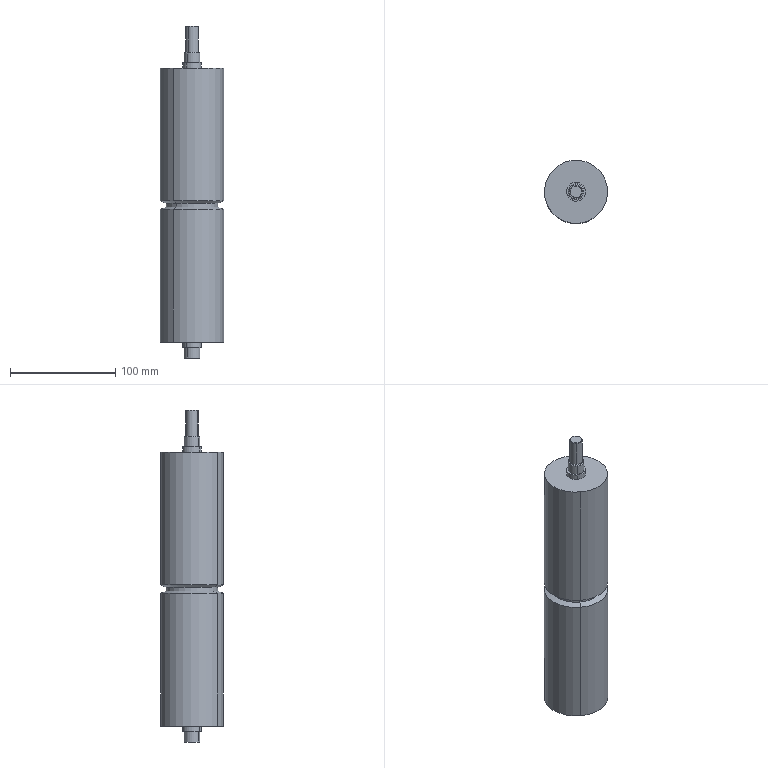Component | SolidWorks | LD101-02--Q1024-Q1-2-1 | 1 solid | 31 faces | box 60 x 60 x 315 mm | volume 738446 mm3 | cylinder 16 | cone 8 | plane 7 | commonest cylinder face diameters 60 x4 18 x4 15 x4 49 x2 12 x2 | material 45
build123d program:
from build123d import *

# Parameters (mm, degrees)
SKETCH1_R           = 30
SKETCH1_R_2         = 25
EXTRUDE_THIN1_DEPTH = 130
BOSS_EXTRUDE1_START = -260
SKETCH2_R           = 25
BOSS_EXTRUDE1_DEPTH = 260
SKETCH3_R           = 9
BOSS_EXTRUDE2_DEPTH = 5
SKETCH5_R           = 7.5
BOSS_EXTRUDE4_DEPTH = 10
BOSS_EXTRUDE5_START = 10
SKETCH6_R           = 7.5
BOSS_EXTRUDE5_DEPTH = 10
CHAMFER4_SIZE       = 0.6
SKETCH7_R           = 6
BOSS_EXTRUDE6_DEPTH = 25
CHAMFER3_SIZE       = 0.6


with BuildPart() as part:
    # Sketch1 → Extrude-Thin1 (new, symmetric)
    with BuildSketch(Plane.XY):
        Circle(SKETCH1_R)
        Circle(SKETCH1_R_2, mode=Mode.SUBTRACT)
    extrude(amount=EXTRUDE_THIN1_DEPTH, both=True)

    # Sketch2 → Boss-Extrude1 (add)
    with BuildSketch(Plane.XY.offset(130).offset(BOSS_EXTRUDE1_START)):
        Circle(SKETCH2_R)
    extrude(amount=BOSS_EXTRUDE1_DEPTH)

    # Sketch3 → Boss-Extrude2 (add)
    with BuildSketch(Plane.XY.offset(130)):
        Circle(SKETCH3_R)
    extrude(amount=BOSS_EXTRUDE2_DEPTH)

    # Mirror2: part across plane


with BuildPart() as part_1:
    add(part.part)
    add(part.part.mirror(Plane.XY))

    # Sketch5 → Boss-Extrude4 (add)
    with BuildSketch(Plane.XY.offset(135)):
        Circle(SKETCH5_R)
    extrude(amount=BOSS_EXTRUDE4_DEPTH)

    # Sketch6 → Boss-Extrude5 (add)
    with BuildSketch(Plane(origin=(0, 0, -135), x_dir=(-1, 0, 0), z_dir=(0, 0, -1)).offset(BOSS_EXTRUDE5_START)):
        with Locations(Location((0, 0, 0), (0, 0, 180))):
            Circle(SKETCH6_R)
    extrude(amount=-BOSS_EXTRUDE5_DEPTH)

    # Chamfer4
    chamfer4_edges = [part_1.edges().sort_by_distance(p)[0] for p in [
        (-7.5, 0, 145),
    ]]
    chamfer(chamfer4_edges, length=CHAMFER4_SIZE)

    # Sketch7 → Boss-Extrude6 (add)
    with BuildSketch(Plane(origin=(0, 0, 145), x_dir=(-1, 0, 0), z_dir=(0, 0, -1))):
        Circle(SKETCH7_R)
    extrude(amount=-BOSS_EXTRUDE6_DEPTH)

    # Chamfer3
    chamfer3_edges = [part_1.edges().sort_by_distance(p)[0] for p in [
        (6, 0, 170),
    ]]
    chamfer(chamfer3_edges, length=CHAMFER3_SIZE)

    # Sketch8 → Cut-Revolve1 (revolve, cut)
    with BuildSketch(Plane(origin=(0, 0, 0), x_dir=(1, 0, 0), z_dir=(0, 1, 0)), mode=Mode.PRIVATE) as cut_revolve1_sk:
        Polygon((-30, 4), (-30, -4), (-30, -4.025), (-24.5, -1.825), (-24.5, 1.825), (-30, 4.025), align=None)
    revolve(cut_revolve1_sk.sketch.rotate(Axis((0, 0, 130), (0, 0, -1)), 180), axis=Axis((0, 0, 130), (0, 0, -1)), mode=Mode.SUBTRACT)


solid = part_1.part

# Placed as in the assembly
solid = solid.moved(Location((371.71, -181.897, 146.257), (0, 0, 0)))
STEP:
#1=COLOUR_RGB('',0.7922,0.8196,0.9333);
#2=FILL_AREA_STYLE_COLOUR('',#1);
#3=FILL_AREA_STYLE('',(#2));
#4=SURFACE_STYLE_FILL_AREA(#3);
#5=SURFACE_SIDE_STYLE('',(#4));
#6=SURFACE_STYLE_USAGE(.BOTH.,#5);
#7=PRESENTATION_STYLE_ASSIGNMENT((#6));
#8=CARTESIAN_POINT('',(13.933,-8.112,5.6));
#9=VERTEX_POINT('',#8);
#10=CARTESIAN_POINT('',(15.336,-6.211,5.6));
#11=VERTEX_POINT('',#10);
#12=CARTESIAN_POINT('',(14.634,-7.161,5.6));
#13=DIRECTION('',(-0.,-0.,1.));
#14=DIRECTION('',(-0.5939,-0.8045,0.));
#15=AXIS2_PLACEMENT_3D('',#12,#13,#14);
#16=CIRCLE('',#15,1.181);
#17=EDGE_CURVE('',#9,#11,#16,.T.);
#18=ORIENTED_EDGE('',*,*,#17,.F.);
#19=CARTESIAN_POINT('',(13.933,-8.112,0.64));
#20=VERTEX_POINT('',#19);
#21=CARTESIAN_POINT('',(13.933,-8.112,10.876));
#22=DIRECTION('',(0.,0.,-1.));
#23=VECTOR('',#22,39.37);
#24=LINE('',#21,#23);
#25=EDGE_CURVE('',#9,#20,#24,.T.);
#26=ORIENTED_EDGE('',*,*,#25,.T.);
#27=CARTESIAN_POINT('',(15.336,-6.211,0.64));
#28=VERTEX_POINT('',#27);
#29=CARTESIAN_POINT('',(14.634,-7.161,0.64));
#30=DIRECTION('',(0.,0.,1.));
#31=DIRECTION('',(-0.5939,-0.8045,0.));
#32=AXIS2_PLACEMENT_3D('',#29,#30,#31);
#33=CIRCLE('',#32,1.181);
#34=EDGE_CURVE('',#20,#28,#33,.T.);
#35=ORIENTED_EDGE('',*,*,#34,.T.);
#36=CARTESIAN_POINT('',(15.336,-6.211,10.876));
#37=DIRECTION('',(0.,0.,-1.));
#38=VECTOR('',#37,39.37);
#39=LINE('',#36,#38);
#40=EDGE_CURVE('',#11,#28,#39,.T.);
#41=ORIENTED_EDGE('',*,*,#40,.F.);
#42=EDGE_LOOP('',(#18,#26,#35,#41));
#43=FACE_OUTER_BOUND('',#42,.T.);
#44=CARTESIAN_POINT('',(14.634,-7.161,10.876));
#45=DIRECTION('',(0.,0.,-1.));
#46=DIRECTION('',(0.5939,0.8045,0.));
#47=AXIS2_PLACEMENT_3D('',#44,#45,#46);
#48=CYLINDRICAL_SURFACE('',#47,1.181);
#49=ADVANCED_FACE('',(#43),#48,.T.);
#50=CARTESIAN_POINT('',(14.845,-6.876,0.4432));
#51=VERTEX_POINT('',#50);
#52=CARTESIAN_POINT('',(14.424,-7.446,0.4432));
#53=VERTEX_POINT('',#52);
#54=CARTESIAN_POINT('',(14.634,-7.161,0.4432));
#55=DIRECTION('',(0.,0.,1.));
#56=DIRECTION('',(-0.5939,-0.8045,0.));
#57=AXIS2_PLACEMENT_3D('',#54,#55,#56);
#58=CIRCLE('',#57,0.3543);
#59=EDGE_CURVE('',#51,#53,#58,.T.);
#60=ORIENTED_EDGE('',*,*,#59,.T.);
#61=CARTESIAN_POINT('',(14.424,-7.446,0.64));
#62=VERTEX_POINT('',#61);
#63=CARTESIAN_POINT('',(14.424,-7.446,0.4432));
#64=DIRECTION('',(0.,0.,1.));
#65=VECTOR('',#64,39.37);
#66=LINE('',#63,#65);
#67=EDGE_CURVE('',#53,#62,#66,.T.);
#68=ORIENTED_EDGE('',*,*,#67,.T.);
#69=CARTESIAN_POINT('',(14.845,-6.876,0.64));
#70=VERTEX_POINT('',#69);
#71=CARTESIAN_POINT('',(14.634,-7.161,0.64));
#72=DIRECTION('',(0.,0.,-1.));
#73=DIRECTION('',(-0.5939,-0.8045,0.));
#74=AXIS2_PLACEMENT_3D('',#71,#72,#73);
#75=CIRCLE('',#74,0.3543);
#76=EDGE_CURVE('',#62,#70,#75,.T.);
#77=ORIENTED_EDGE('',*,*,#76,.T.);
#78=CARTESIAN_POINT('',(14.845,-6.876,0.4432));
#79=DIRECTION('',(0.,0.,1.));
#80=VECTOR('',#79,39.37);
#81=LINE('',#78,#80);
#82=EDGE_CURVE('',#51,#70,#81,.T.);
#83=ORIENTED_EDGE('',*,*,#82,.F.);
#84=EDGE_LOOP('',(#60,#68,#77,#83));
#85=FACE_OUTER_BOUND('',#84,.T.);
#86=CARTESIAN_POINT('',(14.634,-7.161,0.4432));
#87=DIRECTION('',(0.,0.,1.));
#88=DIRECTION('',(0.5939,0.8045,0.));
#89=AXIS2_PLACEMENT_3D('',#86,#87,#88);
#90=CYLINDRICAL_SURFACE('',#89,0.3543);
#91=ADVANCED_FACE('',(#85),#90,.T.);
#92=CARTESIAN_POINT('',(14.81,-6.924,0.04947));
#93=VERTEX_POINT('',#92);
#94=CARTESIAN_POINT('',(14.459,-7.399,0.04947));
#95=VERTEX_POINT('',#94);
#96=CARTESIAN_POINT('',(14.634,-7.161,0.04947));
#97=DIRECTION('',(0.,0.,-1.));
#98=DIRECTION('',(0.5939,0.8045,0.));
#99=AXIS2_PLACEMENT_3D('',#96,#97,#98);
#100=CIRCLE('',#99,0.2953);
#101=EDGE_CURVE('',#93,#95,#100,.T.);
#102=ORIENTED_EDGE('',*,*,#101,.F.);
#103=CARTESIAN_POINT('',(14.81,-6.924,0.4432));
#104=VERTEX_POINT('',#103);
#105=CARTESIAN_POINT('',(14.81,-6.924,0.04947));
#106=DIRECTION('',(0.,0.,1.));
#107=VECTOR('',#106,39.37);
#108=LINE('',#105,#107);
#109=EDGE_CURVE('',#93,#104,#108,.T.);
#110=ORIENTED_EDGE('',*,*,#109,.T.);
#111=CARTESIAN_POINT('',(14.459,-7.399,0.4432));
#112=VERTEX_POINT('',#111);
#113=CARTESIAN_POINT('',(14.634,-7.161,0.4432));
#114=DIRECTION('',(0.,0.,-1.));
#115=DIRECTION('',(0.5939,0.8045,0.));
#116=AXIS2_PLACEMENT_3D('',#113,#114,#115);
#117=CIRCLE('',#116,0.2953);
#118=EDGE_CURVE('',#104,#112,#117,.T.);
#119=ORIENTED_EDGE('',*,*,#118,.T.);
#120=CARTESIAN_POINT('',(14.459,-7.399,0.04947));
#121=DIRECTION('',(0.,0.,1.));
#122=VECTOR('',#121,39.37);
#123=LINE('',#120,#122);
#124=EDGE_CURVE('',#95,#112,#123,.T.);
#125=ORIENTED_EDGE('',*,*,#124,.F.);
#126=EDGE_LOOP('',(#102,#110,#119,#125));
#127=FACE_OUTER_BOUND('',#126,.T.);
#128=CARTESIAN_POINT('',(14.634,-7.161,0.04947));
#129=DIRECTION('',(0.,0.,1.));
#130=DIRECTION('',(-0.5939,-0.8045,0.));
#131=AXIS2_PLACEMENT_3D('',#128,#129,#130);
#132=CYLINDRICAL_SURFACE('',#131,0.2953);
#133=ADVANCED_FACE('',(#127),#132,.T.);
#134=CARTESIAN_POINT('',(14.061,-7.937,5.83));
#135=VERTEX_POINT('',#134);
#136=CARTESIAN_POINT('',(15.207,-6.385,5.83));
#137=VERTEX_POINT('',#136);
#138=CARTESIAN_POINT('',(14.634,-7.161,5.83));
#139=DIRECTION('',(-0.,-0.,1.));
#140=DIRECTION('',(-0.5939,-0.8045,0.));
#141=AXIS2_PLACEMENT_3D('',#138,#139,#140);
#142=CIRCLE('',#141,0.9646);
#143=EDGE_CURVE('',#135,#137,#142,.T.);
#144=ORIENTED_EDGE('',*,*,#143,.T.);
#145=CARTESIAN_POINT('',(15.336,-6.211,5.917));
#146=VERTEX_POINT('',#145);
#147=CARTESIAN_POINT('',(15.336,-6.211,5.917));
#148=DIRECTION('',(0.5514,0.747,0.3714));
#149=VECTOR('',#148,39.37);
#150=LINE('',#147,#149);
#151=EDGE_CURVE('',#137,#146,#150,.T.);
#152=ORIENTED_EDGE('',*,*,#151,.T.);
#153=CARTESIAN_POINT('',(13.933,-8.112,5.917));
#154=VERTEX_POINT('',#153);
#155=CARTESIAN_POINT('',(14.634,-7.161,5.917));
#156=DIRECTION('',(-0.,-0.,1.));
#157=DIRECTION('',(-0.5939,-0.8045,0.));
#158=AXIS2_PLACEMENT_3D('',#155,#156,#157);
#159=CIRCLE('',#158,1.181);
#160=EDGE_CURVE('',#154,#146,#159,.T.);
#161=ORIENTED_EDGE('',*,*,#160,.F.);
#162=CARTESIAN_POINT('',(13.933,-8.112,5.917));
#163=DIRECTION('',(-0.5514,-0.747,0.3714));
#164=VECTOR('',#163,39.37);
#165=LINE('',#162,#164);
#166=EDGE_CURVE('',#135,#154,#165,.T.);
#167=ORIENTED_EDGE('',*,*,#166,.F.);
#168=EDGE_LOOP('',(#144,#152,#161,#167));
#169=FACE_OUTER_BOUND('',#168,.T.);
#170=CARTESIAN_POINT('',(14.634,-7.161,5.917));
#171=DIRECTION('',(-0.,-0.,1.));
#172=DIRECTION('',(-0.5939,-0.8045,0.));
#173=AXIS2_PLACEMENT_3D('',#170,#171,#172);
#174=CONICAL_SURFACE('',#173,1.181,1.19);
#175=ADVANCED_FACE('',(#169),#174,.T.);
#176=CARTESIAN_POINT('',(14.061,-7.937,5.686));
#177=VERTEX_POINT('',#176);
#178=CARTESIAN_POINT('',(15.207,-6.385,5.686));
#179=VERTEX_POINT('',#178);
#180=CARTESIAN_POINT('',(14.634,-7.161,5.686));
#181=DIRECTION('',(-0.,-0.,1.));
#182=DIRECTION('',(-0.5939,-0.8045,0.));
#183=AXIS2_PLACEMENT_3D('',#180,#181,#182);
#184=CIRCLE('',#183,0.9646);
#185=EDGE_CURVE('',#177,#179,#184,.T.);
#186=ORIENTED_EDGE('',*,*,#185,.T.);
#187=CARTESIAN_POINT('',(15.207,-6.385,10.876));
#188=DIRECTION('',(-0.,-0.,1.));
#189=VECTOR('',#188,39.37);
#190=LINE('',#187,#189);
#191=EDGE_CURVE('',#179,#137,#190,.T.);
#192=ORIENTED_EDGE('',*,*,#191,.T.);
#193=ORIENTED_EDGE('',*,*,#143,.F.);
#194=CARTESIAN_POINT('',(14.061,-7.937,10.876));
#195=DIRECTION('',(-0.,-0.,1.));
#196=VECTOR('',#195,39.37);
#197=LINE('',#194,#196);
#198=EDGE_CURVE('',#177,#135,#197,.T.);
#199=ORIENTED_EDGE('',*,*,#198,.F.);
#200=EDGE_LOOP('',(#186,#192,#193,#199));
#201=FACE_OUTER_BOUND('',#200,.T.);
#202=CARTESIAN_POINT('',(14.634,-7.161,10.876));
#203=DIRECTION('',(-0.,-0.,1.));
#204=DIRECTION('',(-0.5939,-0.8045,0.));
#205=AXIS2_PLACEMENT_3D('',#202,#203,#204);
#206=CYLINDRICAL_SURFACE('',#205,0.9646);
#207=ADVANCED_FACE('',(#201),#206,.T.);
#208=ORIENTED_EDGE('',*,*,#185,.F.);
#209=CARTESIAN_POINT('',(14.061,-7.937,5.686));
#210=DIRECTION('',(-0.5514,-0.747,-0.3714));
#211=VECTOR('',#210,39.37);
#212=LINE('',#209,#211);
#213=EDGE_CURVE('',#177,#9,#212,.T.);
#214=ORIENTED_EDGE('',*,*,#213,.T.);
#215=ORIENTED_EDGE('',*,*,#17,.T.);
#216=CARTESIAN_POINT('',(15.207,-6.385,5.686));
#217=DIRECTION('',(0.5514,0.747,-0.3714));
#218=VECTOR('',#217,39.37);
#219=LINE('',#216,#218);
#220=EDGE_CURVE('',#179,#11,#219,.T.);
#221=ORIENTED_EDGE('',*,*,#220,.F.);
#222=EDGE_LOOP('',(#208,#214,#215,#221));
#223=FACE_OUTER_BOUND('',#222,.T.);
#224=CARTESIAN_POINT('',(14.634,-7.161,5.686));
#225=DIRECTION('',(0.,0.,-1.));
#226=DIRECTION('',(0.5939,0.8045,0.));
#227=AXIS2_PLACEMENT_3D('',#224,#225,#226);
#228=CONICAL_SURFACE('',#227,0.9646,1.19);
#229=ADVANCED_FACE('',(#223),#228,.T.);
#230=CARTESIAN_POINT('',(14.508,-7.332,12.451));
#231=VERTEX_POINT('',#230);
#232=CARTESIAN_POINT('',(14.761,-6.99,12.451));
#233=VERTEX_POINT('',#232);
#234=CARTESIAN_POINT('',(14.634,-7.161,12.451));
#235=DIRECTION('',(0.,0.,1.));
#236=DIRECTION('',(0.5939,0.8045,0.));
#237=AXIS2_PLACEMENT_3D('',#234,#235,#236);
#238=CIRCLE('',#237,0.2126);
#239=EDGE_CURVE('',#231,#233,#238,.T.);
#240=ORIENTED_EDGE('',*,*,#239,.F.);
#241=CARTESIAN_POINT('',(14.494,-7.351,12.427));
#242=VERTEX_POINT('',#241);
#243=CARTESIAN_POINT('',(14.494,-7.351,12.427));
#244=DIRECTION('',(-0.4199,-0.5689,-0.7071));
#245=VECTOR('',#244,39.37);
#246=LINE('',#243,#245);
#247=EDGE_CURVE('',#231,#242,#246,.T.);
#248=ORIENTED_EDGE('',*,*,#247,.T.);
#249=CARTESIAN_POINT('',(14.775,-6.971,12.427));
#250=VERTEX_POINT('',#249);
#251=CARTESIAN_POINT('',(14.634,-7.161,12.427));
#252=DIRECTION('',(0.,0.,-1.));
#253=DIRECTION('',(0.5939,0.8045,0.));
#254=AXIS2_PLACEMENT_3D('',#251,#252,#253);
#255=CIRCLE('',#254,0.2362);
#256=EDGE_CURVE('',#250,#242,#255,.T.);
#257=ORIENTED_EDGE('',*,*,#256,.F.);
#258=CARTESIAN_POINT('',(14.775,-6.971,12.427));
#259=DIRECTION('',(0.4199,0.5689,-0.7071));
#260=VECTOR('',#259,39.37);
#261=LINE('',#258,#260);
#262=EDGE_CURVE('',#233,#250,#261,.T.);
#263=ORIENTED_EDGE('',*,*,#262,.F.);
#264=EDGE_LOOP('',(#240,#248,#257,#263));
#265=FACE_OUTER_BOUND('',#264,.T.);
#266=CARTESIAN_POINT('',(14.634,-7.161,12.427));
#267=DIRECTION('',(0.,0.,-1.));
#268=DIRECTION('',(0.5939,0.8045,0.));
#269=AXIS2_PLACEMENT_3D('',#266,#267,#268);
#270=CONICAL_SURFACE('',#269,0.2362,0.7854);
#271=ADVANCED_FACE('',(#265),#270,.T.);
#272=ORIENTED_EDGE('',*,*,#256,.T.);
#273=CARTESIAN_POINT('',(14.494,-7.351,11.467));
#274=VERTEX_POINT('',#273);
#275=CARTESIAN_POINT('',(14.494,-7.351,12.451));
#276=DIRECTION('',(0.,0.,-1.));
#277=VECTOR('',#276,39.37);
#278=LINE('',#275,#277);
#279=EDGE_CURVE('',#242,#274,#278,.T.);
#280=ORIENTED_EDGE('',*,*,#279,.T.);
#281=CARTESIAN_POINT('',(14.775,-6.971,11.467));
#282=VERTEX_POINT('',#281);
#283=CARTESIAN_POINT('',(14.634,-7.161,11.467));
#284=DIRECTION('',(0.,0.,1.));
#285=DIRECTION('',(-0.5939,-0.8045,0.));
#286=AXIS2_PLACEMENT_3D('',#283,#284,#285);
#287=CIRCLE('',#286,0.2362);
#288=EDGE_CURVE('',#274,#282,#287,.T.);
#289=ORIENTED_EDGE('',*,*,#288,.T.);
#290=CARTESIAN_POINT('',(14.775,-6.971,12.451));
#291=DIRECTION('',(0.,0.,-1.));
#292=VECTOR('',#291,39.37);
#293=LINE('',#290,#292);
#294=EDGE_CURVE('',#250,#282,#293,.T.);
#295=ORIENTED_EDGE('',*,*,#294,.F.);
#296=EDGE_LOOP('',(#272,#280,#289,#295));
#297=FACE_OUTER_BOUND('',#296,.T.);
#298=CARTESIAN_POINT('',(14.634,-7.161,12.451));
#299=DIRECTION('',(0.,0.,-1.));
#300=DIRECTION('',(0.5939,0.8045,0.));
#301=AXIS2_PLACEMENT_3D('',#298,#299,#300);
#302=CYLINDRICAL_SURFACE('',#301,0.2362);
#303=ADVANCED_FACE('',(#297),#302,.T.);
#304=CARTESIAN_POINT('',(14.473,-7.38,11.467));
#305=VERTEX_POINT('',#304);
#306=CARTESIAN_POINT('',(14.796,-6.943,11.467));
#307=VERTEX_POINT('',#306);
#308=CARTESIAN_POINT('',(14.634,-7.161,11.467));
#309=DIRECTION('',(0.,0.,1.));
#310=DIRECTION('',(-0.5939,-0.8045,0.));
#311=AXIS2_PLACEMENT_3D('',#308,#309,#310);
#312=CIRCLE('',#311,0.2717);
#313=EDGE_CURVE('',#305,#307,#312,.T.);
#314=ORIENTED_EDGE('',*,*,#313,.F.);
#315=CARTESIAN_POINT('',(14.459,-7.399,11.443));
#316=VERTEX_POINT('',#315);
#317=CARTESIAN_POINT('',(14.473,-7.38,11.467));
#318=DIRECTION('',(-0.4199,-0.5689,-0.7071));
#319=VECTOR('',#318,39.37);
#320=LINE('',#317,#319);
#321=EDGE_CURVE('',#305,#316,#320,.T.);
#322=ORIENTED_EDGE('',*,*,#321,.T.);
#323=CARTESIAN_POINT('',(14.81,-6.924,11.443));
#324=VERTEX_POINT('',#323);
#325=CARTESIAN_POINT('',(14.634,-7.161,11.443));
#326=DIRECTION('',(0.,0.,-1.));
#327=DIRECTION('',(-0.5939,-0.8045,0.));
#328=AXIS2_PLACEMENT_3D('',#325,#326,#327);
#329=CIRCLE('',#328,0.2953);
#330=EDGE_CURVE('',#324,#316,#329,.T.);
#331=ORIENTED_EDGE('',*,*,#330,.F.);
#332=CARTESIAN_POINT('',(14.796,-6.943,11.467));
#333=DIRECTION('',(0.4199,0.5689,-0.7071));
#334=VECTOR('',#333,39.37);
#335=LINE('',#332,#334);
#336=EDGE_CURVE('',#307,#324,#335,.T.);
#337=ORIENTED_EDGE('',*,*,#336,.F.);
#338=EDGE_LOOP('',(#314,#322,#331,#337));
#339=FACE_OUTER_BOUND('',#338,.T.);
#340=CARTESIAN_POINT('',(14.634,-7.161,11.467));
#341=DIRECTION('',(0.,0.,-1.));
#342=DIRECTION('',(0.5939,0.8045,0.));
#343=AXIS2_PLACEMENT_3D('',#340,#341,#342);
#344=CONICAL_SURFACE('',#343,0.2717,0.7854);
#345=ADVANCED_FACE('',(#339),#344,.T.);
#346=ORIENTED_EDGE('',*,*,#330,.T.);
#347=CARTESIAN_POINT('',(14.459,-7.399,11.073));
#348=VERTEX_POINT('',#347);
#349=CARTESIAN_POINT('',(14.459,-7.399,11.467));
#350=DIRECTION('',(0.,0.,-1.));
#351=VECTOR('',#350,39.37);
#352=LINE('',#349,#351);
#353=EDGE_CURVE('',#316,#348,#352,.T.);
#354=ORIENTED_EDGE('',*,*,#353,.T.);
#355=CARTESIAN_POINT('',(14.81,-6.924,11.073));
#356=VERTEX_POINT('',#355);
#357=CARTESIAN_POINT('',(14.634,-7.161,11.073));
#358=DIRECTION('',(0.,0.,1.));
#359=DIRECTION('',(-0.5939,-0.8045,0.));
#360=AXIS2_PLACEMENT_3D('',#357,#358,#359);
#361=CIRCLE('',#360,0.2953);
#362=EDGE_CURVE('',#348,#356,#361,.T.);
#363=ORIENTED_EDGE('',*,*,#362,.T.);
#364=CARTESIAN_POINT('',(14.81,-6.924,11.467));
#365=DIRECTION('',(0.,0.,-1.));
#366=VECTOR('',#365,39.37);
#367=LINE('',#364,#366);
#368=EDGE_CURVE('',#324,#356,#367,.T.);
#369=ORIENTED_EDGE('',*,*,#368,.F.);
#370=EDGE_LOOP('',(#346,#354,#363,#369));
#371=FACE_OUTER_BOUND('',#370,.T.);
#372=CARTESIAN_POINT('',(14.634,-7.161,11.467));
#373=DIRECTION('',(0.,0.,-1.));
#374=DIRECTION('',(0.5939,0.8045,0.));
#375=AXIS2_PLACEMENT_3D('',#372,#373,#374);
#376=CYLINDRICAL_SURFACE('',#375,0.2953);
#377=ADVANCED_FACE('',(#371),#376,.T.);
#378=CARTESIAN_POINT('',(14.424,-7.446,11.073));
#379=VERTEX_POINT('',#378);
#380=CARTESIAN_POINT('',(14.845,-6.876,11.073));
#381=VERTEX_POINT('',#380);
#382=CARTESIAN_POINT('',(14.634,-7.161,11.073));
#383=DIRECTION('',(0.,0.,1.));
#384=DIRECTION('',(-0.5939,-0.8045,0.));
#385=AXIS2_PLACEMENT_3D('',#382,#383,#384);
#386=CIRCLE('',#385,0.3543);
#387=EDGE_CURVE('',#379,#381,#386,.T.);
#388=ORIENTED_EDGE('',*,*,#387,.F.);
#389=CARTESIAN_POINT('',(14.424,-7.446,10.876));
#390=VERTEX_POINT('',#389);
#391=CARTESIAN_POINT('',(14.424,-7.446,11.073));
#392=DIRECTION('',(0.,0.,-1.));
#393=VECTOR('',#392,39.37);
#394=LINE('',#391,#393);
#395=EDGE_CURVE('',#379,#390,#394,.T.);
#396=ORIENTED_EDGE('',*,*,#395,.T.);
#397=CARTESIAN_POINT('',(14.845,-6.876,10.876));
#398=VERTEX_POINT('',#397);
#399=CARTESIAN_POINT('',(14.634,-7.161,10.876));
#400=DIRECTION('',(0.,0.,1.));
#401=DIRECTION('',(-0.5939,-0.8045,0.));
#402=AXIS2_PLACEMENT_3D('',#399,#400,#401);
#403=CIRCLE('',#402,0.3543);
#404=EDGE_CURVE('',#390,#398,#403,.T.);
#405=ORIENTED_EDGE('',*,*,#404,.T.);
#406=CARTESIAN_POINT('',(14.845,-6.876,11.073));
#407=DIRECTION('',(0.,0.,-1.));
#408=VECTOR('',#407,39.37);
#409=LINE('',#406,#408);
#410=EDGE_CURVE('',#381,#398,#409,.T.);
#411=ORIENTED_EDGE('',*,*,#410,.F.);
#412=EDGE_LOOP('',(#388,#396,#405,#411));
#413=FACE_OUTER_BOUND('',#412,.T.);
#414=CARTESIAN_POINT('',(14.634,-7.161,11.073));
#415=DIRECTION('',(0.,0.,-1.));
#416=DIRECTION('',(0.5939,0.8045,0.));
#417=AXIS2_PLACEMENT_3D('',#414,#415,#416);
#418=CYLINDRICAL_SURFACE('',#417,0.3543);
#419=ADVANCED_FACE('',(#413),#418,.T.);
#420=CARTESIAN_POINT('',(13.933,-8.112,10.876));
#421=VERTEX_POINT('',#420);
#422=CARTESIAN_POINT('',(15.336,-6.211,10.876));
#423=VERTEX_POINT('',#422);
#424=CARTESIAN_POINT('',(14.634,-7.161,10.876));
#425=DIRECTION('',(0.,0.,1.));
#426=DIRECTION('',(-0.5939,-0.8045,0.));
#427=AXIS2_PLACEMENT_3D('',#424,#425,#426);
#428=CIRCLE('',#427,1.181);
#429=EDGE_CURVE('',#421,#423,#428,.T.);
#430=ORIENTED_EDGE('',*,*,#429,.F.);
#431=CARTESIAN_POINT('',(13.933,-8.112,10.876));
#432=DIRECTION('',(0.,0.,-1.));
#433=VECTOR('',#432,39.37);
#434=LINE('',#431,#433);
#435=EDGE_CURVE('',#421,#154,#434,.T.);
#436=ORIENTED_EDGE('',*,*,#435,.T.);
#437=ORIENTED_EDGE('',*,*,#160,.T.);
#438=CARTESIAN_POINT('',(15.336,-6.211,10.876));
#439=DIRECTION('',(0.,0.,-1.));
#440=VECTOR('',#439,39.37);
#441=LINE('',#438,#440);
#442=EDGE_CURVE('',#423,#146,#441,.T.);
#443=ORIENTED_EDGE('',*,*,#442,.F.);
#444=EDGE_LOOP('',(#430,#436,#437,#443));
#445=FACE_OUTER_BOUND('',#444,.T.);
#446=CARTESIAN_POINT('',(14.634,-7.161,10.876));
#447=DIRECTION('',(0.,0.,-1.));
#448=DIRECTION('',(0.5939,0.8045,0.));
#449=AXIS2_PLACEMENT_3D('',#446,#447,#448);
#450=CYLINDRICAL_SURFACE('',#449,1.181);
#451=ADVANCED_FACE('',(#445),#450,.T.);
#452=ORIENTED_EDGE('',*,*,#435,.F.);
#453=CARTESIAN_POINT('',(14.634,-7.161,10.876));
#454=DIRECTION('',(0.,0.,1.));
#455=DIRECTION('',(-0.5939,-0.8045,0.));
#456=AXIS2_PLACEMENT_3D('',#453,#454,#455);
#457=CIRCLE('',#456,1.181);
#458=EDGE_CURVE('',#423,#421,#457,.T.);
#459=ORIENTED_EDGE('',*,*,#458,.F.);
#460=ORIENTED_EDGE('',*,*,#442,.T.);
#461=CARTESIAN_POINT('',(14.634,-7.161,5.917));
#462=DIRECTION('',(-0.,-0.,1.));
#463=DIRECTION('',(-0.5939,-0.8045,0.));
#464=AXIS2_PLACEMENT_3D('',#461,#462,#463);
#465=CIRCLE('',#464,1.181);
#466=EDGE_CURVE('',#146,#154,#465,.T.);
#467=ORIENTED_EDGE('',*,*,#466,.T.);
#468=EDGE_LOOP('',(#452,#459,#460,#467));
#469=FACE_OUTER_BOUND('',#468,.T.);
#470=CARTESIAN_POINT('',(14.634,-7.161,10.876));
#471=DIRECTION('',(0.,0.,-1.));
#472=DIRECTION('',(0.5939,0.8045,0.));
#473=AXIS2_PLACEMENT_3D('',#470,#471,#472);
#474=CYLINDRICAL_SURFACE('',#473,1.181);
#475=ADVANCED_FACE('',(#469),#474,.T.);
#476=CARTESIAN_POINT('',(14.634,-7.161,11.073));
#477=DIRECTION('',(0.,0.,1.));
#478=DIRECTION('',(-0.5939,-0.8045,0.));
#479=AXIS2_PLACEMENT_3D('',#476,#477,#478);
#480=CIRCLE('',#479,0.3543);
#481=EDGE_CURVE('',#381,#379,#480,.T.);
#482=ORIENTED_EDGE('',*,*,#481,.T.);
#483=ORIENTED_EDGE('',*,*,#387,.T.);
#484=EDGE_LOOP('',(#482,#483));
#485=FACE_OUTER_BOUND('',#484,.T.);
#486=CARTESIAN_POINT('',(14.634,-7.161,11.073));
#487=DIRECTION('',(0.,0.,1.));
#488=DIRECTION('',(-0.5939,-0.8045,0.));
#489=AXIS2_PLACEMENT_3D('',#486,#487,#488);
#490=CIRCLE('',#489,0.2953);
#491=EDGE_CURVE('',#356,#348,#490,.T.);
#492=ORIENTED_EDGE('',*,*,#491,.F.);
#493=ORIENTED_EDGE('',*,*,#362,.F.);
#494=EDGE_LOOP('',(#492,#493));
#495=FACE_BOUND('',#494,.T.);
#496=CARTESIAN_POINT('',(14.634,-7.161,11.073));
#497=DIRECTION('',(0.,0.,1.));
#498=DIRECTION('',(-0.5939,-0.8045,0.));
#499=AXIS2_PLACEMENT_3D('',#496,#497,#498);
#500=PLANE('',#499);
#501=ADVANCED_FACE('',(#485,#495),#500,.T.);
#502=ORIENTED_EDGE('',*,*,#458,.T.);
#503=ORIENTED_EDGE('',*,*,#429,.T.);
#504=EDGE_LOOP('',(#502,#503));
#505=FACE_OUTER_BOUND('',#504,.T.);
#506=CARTESIAN_POINT('',(14.634,-7.161,10.876));
#507=DIRECTION('',(0.,0.,1.));
#508=DIRECTION('',(-0.5939,-0.8045,0.));
#509=AXIS2_PLACEMENT_3D('',#506,#507,#508);
#510=CIRCLE('',#509,0.3543);
#511=EDGE_CURVE('',#398,#390,#510,.T.);
#512=ORIENTED_EDGE('',*,*,#511,.F.);
#513=ORIENTED_EDGE('',*,*,#404,.F.);
#514=EDGE_LOOP('',(#512,#513));
#515=FACE_BOUND('',#514,.T.);
#516=CARTESIAN_POINT('',(14.634,-7.161,10.876));
#517=DIRECTION('',(0.,0.,1.));
#518=DIRECTION('',(-0.5939,-0.8045,0.));
#519=AXIS2_PLACEMENT_3D('',#516,#517,#518);
#520=PLANE('',#519);
#521=ADVANCED_FACE('',(#505,#515),#520,.T.);
#522=ORIENTED_EDGE('',*,*,#395,.F.);
#523=ORIENTED_EDGE('',*,*,#481,.F.);
#524=ORIENTED_EDGE('',*,*,#410,.T.);
#525=ORIENTED_EDGE('',*,*,#511,.T.);
#526=EDGE_LOOP('',(#522,#523,#524,#525));
#527=FACE_OUTER_BOUND('',#526,.T.);
#528=CARTESIAN_POINT('',(14.634,-7.161,11.073));
#529=DIRECTION('',(0.,0.,-1.));
#530=DIRECTION('',(0.5939,0.8045,0.));
#531=AXIS2_PLACEMENT_3D('',#528,#529,#530);
#532=CYLINDRICAL_SURFACE('',#531,0.3543);
#533=ADVANCED_FACE('',(#527),#532,.T.);
#534=ORIENTED_EDGE('',*,*,#353,.F.);
#535=CARTESIAN_POINT('',(14.634,-7.161,11.443));
#536=DIRECTION('',(0.,0.,-1.));
#537=DIRECTION('',(-0.5939,-0.8045,0.));
#538=AXIS2_PLACEMENT_3D('',#535,#536,#537);
#539=CIRCLE('',#538,0.2953);
#540=EDGE_CURVE('',#316,#324,#539,.T.);
#541=ORIENTED_EDGE('',*,*,#540,.T.);
#542=ORIENTED_EDGE('',*,*,#368,.T.);
#543=ORIENTED_EDGE('',*,*,#491,.T.);
#544=EDGE_LOOP('',(#534,#541,#542,#543));
#545=FACE_OUTER_BOUND('',#544,.T.);
#546=CARTESIAN_POINT('',(14.634,-7.161,11.467));
#547=DIRECTION('',(0.,0.,-1.));
#548=DIRECTION('',(0.5939,0.8045,0.));
#549=AXIS2_PLACEMENT_3D('',#546,#547,#548);
#550=CYLINDRICAL_SURFACE('',#549,0.2953);
#551=ADVANCED_FACE('',(#545),#550,.T.);
#552=CARTESIAN_POINT('',(14.634,-7.161,11.467));
#553=DIRECTION('',(0.,0.,1.));
#554=DIRECTION('',(-0.5939,-0.8045,0.));
#555=AXIS2_PLACEMENT_3D('',#552,#553,#554);
#556=CIRCLE('',#555,0.2362);
#557=EDGE_CURVE('',#282,#274,#556,.T.);
#558=ORIENTED_EDGE('',*,*,#557,.F.);
#559=ORIENTED_EDGE('',*,*,#288,.F.);
#560=EDGE_LOOP('',(#558,#559));
#561=FACE_BOUND('',#560,.T.);
#562=CARTESIAN_POINT('',(14.634,-7.161,11.467));
#563=DIRECTION('',(0.,0.,1.));
#564=DIRECTION('',(-0.5939,-0.8045,0.));
#565=AXIS2_PLACEMENT_3D('',#562,#563,#564);
#566=CIRCLE('',#565,0.2717);
#567=EDGE_CURVE('',#307,#305,#566,.T.);
#568=ORIENTED_EDGE('',*,*,#567,.T.);
#569=ORIENTED_EDGE('',*,*,#313,.T.);
#570=EDGE_LOOP('',(#568,#569));
#571=FACE_OUTER_BOUND('',#570,.T.);
#572=CARTESIAN_POINT('',(14.634,-7.161,11.467));
#573=DIRECTION('',(0.,0.,1.));
#574=DIRECTION('',(-0.5939,-0.8045,0.));
#575=AXIS2_PLACEMENT_3D('',#572,#573,#574);
#576=PLANE('',#575);
#577=ADVANCED_FACE('',(#561,#571),#576,.T.);
#578=ORIENTED_EDGE('',*,*,#321,.F.);
#579=ORIENTED_EDGE('',*,*,#567,.F.);
#580=ORIENTED_EDGE('',*,*,#336,.T.);
#581=ORIENTED_EDGE('',*,*,#540,.F.);
#582=EDGE_LOOP('',(#578,#579,#580,#581));
#583=FACE_OUTER_BOUND('',#582,.T.);
#584=CARTESIAN_POINT('',(14.634,-7.161,11.467));
#585=DIRECTION('',(0.,0.,-1.));
#586=DIRECTION('',(0.5939,0.8045,0.));
#587=AXIS2_PLACEMENT_3D('',#584,#585,#586);
#588=CONICAL_SURFACE('',#587,0.2717,0.7854);
#589=ADVANCED_FACE('',(#583),#588,.T.);
#590=ORIENTED_EDGE('',*,*,#279,.F.);
#591=CARTESIAN_POINT('',(14.634,-7.161,12.427));
#592=DIRECTION('',(0.,0.,-1.));
#593=DIRECTION('',(0.5939,0.8045,0.));
#594=AXIS2_PLACEMENT_3D('',#591,#592,#593);
#595=CIRCLE('',#594,0.2362);
#596=EDGE_CURVE('',#242,#250,#595,.T.);
#597=ORIENTED_EDGE('',*,*,#596,.T.);
#598=ORIENTED_EDGE('',*,*,#294,.T.);
#599=ORIENTED_EDGE('',*,*,#557,.T.);
#600=EDGE_LOOP('',(#590,#597,#598,#599));
#601=FACE_OUTER_BOUND('',#600,.T.);
#602=CARTESIAN_POINT('',(14.634,-7.161,12.451));
#603=DIRECTION('',(0.,0.,-1.));
#604=DIRECTION('',(0.5939,0.8045,0.));
#605=AXIS2_PLACEMENT_3D('',#602,#603,#604);
#606=CYLINDRICAL_SURFACE('',#605,0.2362);
#607=ADVANCED_FACE('',(#601),#606,.T.);
#608=CARTESIAN_POINT('',(14.634,-7.161,12.451));
#609=DIRECTION('',(0.,0.,1.));
#610=DIRECTION('',(0.5939,0.8045,0.));
#611=AXIS2_PLACEMENT_3D('',#608,#609,#610);
#612=CIRCLE('',#611,0.2126);
#613=EDGE_CURVE('',#233,#231,#612,.T.);
#614=ORIENTED_EDGE('',*,*,#613,.T.);
#615=ORIENTED_EDGE('',*,*,#239,.T.);
#616=EDGE_LOOP('',(#614,#615));
#617=FACE_OUTER_BOUND('',#616,.T.);
#618=CARTESIAN_POINT('',(14.634,-7.161,12.451));
#619=DIRECTION('',(0.,0.,-1.));
#620=DIRECTION('',(0.5939,0.8045,0.));
#621=AXIS2_PLACEMENT_3D('',#618,#619,#620);
#622=PLANE('',#621);
#623=ADVANCED_FACE('',(#617),#622,.F.);
#624=ORIENTED_EDGE('',*,*,#247,.F.);
#625=ORIENTED_EDGE('',*,*,#613,.F.);
#626=ORIENTED_EDGE('',*,*,#262,.T.);
#627=ORIENTED_EDGE('',*,*,#596,.F.);
#628=EDGE_LOOP('',(#624,#625,#626,#627));
#629=FACE_OUTER_BOUND('',#628,.T.);
#630=CARTESIAN_POINT('',(14.634,-7.161,12.427));
#631=DIRECTION('',(0.,0.,-1.));
#632=DIRECTION('',(0.5939,0.8045,0.));
#633=AXIS2_PLACEMENT_3D('',#630,#631,#632);
#634=CONICAL_SURFACE('',#633,0.2362,0.7854);
#635=ADVANCED_FACE('',(#629),#634,.T.);
#636=ORIENTED_EDGE('',*,*,#213,.F.);
#637=CARTESIAN_POINT('',(14.634,-7.161,5.686));
#638=DIRECTION('',(-0.,-0.,1.));
#639=DIRECTION('',(-0.5939,-0.8045,0.));
#640=AXIS2_PLACEMENT_3D('',#637,#638,#639);
#641=CIRCLE('',#640,0.9646);
#642=EDGE_CURVE('',#179,#177,#641,.T.);
#643=ORIENTED_EDGE('',*,*,#642,.F.);
#644=ORIENTED_EDGE('',*,*,#220,.T.);
#645=CARTESIAN_POINT('',(14.634,-7.161,5.6));
#646=DIRECTION('',(-0.,-0.,1.));
#647=DIRECTION('',(-0.5939,-0.8045,0.));
#648=AXIS2_PLACEMENT_3D('',#645,#646,#647);
#649=CIRCLE('',#648,1.181);
#650=EDGE_CURVE('',#11,#9,#649,.T.);
#651=ORIENTED_EDGE('',*,*,#650,.T.);
#652=EDGE_LOOP('',(#636,#643,#644,#651));
#653=FACE_OUTER_BOUND('',#652,.T.);
#654=CARTESIAN_POINT('',(14.634,-7.161,5.686));
#655=DIRECTION('',(0.,0.,-1.));
#656=DIRECTION('',(0.5939,0.8045,0.));
#657=AXIS2_PLACEMENT_3D('',#654,#655,#656);
#658=CONICAL_SURFACE('',#657,0.9646,1.19);
#659=ADVANCED_FACE('',(#653),#658,.T.);
#660=ORIENTED_EDGE('',*,*,#191,.F.);
#661=ORIENTED_EDGE('',*,*,#642,.T.);
#662=ORIENTED_EDGE('',*,*,#198,.T.);
#663=CARTESIAN_POINT('',(14.634,-7.161,5.83));
#664=DIRECTION('',(-0.,-0.,1.));
#665=DIRECTION('',(-0.5939,-0.8045,0.));
#666=AXIS2_PLACEMENT_3D('',#663,#664,#665);
#667=CIRCLE('',#666,0.9646);
#668=EDGE_CURVE('',#137,#135,#667,.T.);
#669=ORIENTED_EDGE('',*,*,#668,.F.);
#670=EDGE_LOOP('',(#660,#661,#662,#669));
#671=FACE_OUTER_BOUND('',#670,.T.);
#672=CARTESIAN_POINT('',(14.634,-7.161,10.876));
#673=DIRECTION('',(-0.,-0.,1.));
#674=DIRECTION('',(-0.5939,-0.8045,0.));
#675=AXIS2_PLACEMENT_3D('',#672,#673,#674);
#676=CYLINDRICAL_SURFACE('',#675,0.9646);
#677=ADVANCED_FACE('',(#671),#676,.T.);
#678=ORIENTED_EDGE('',*,*,#151,.F.);
#679=ORIENTED_EDGE('',*,*,#668,.T.);
#680=ORIENTED_EDGE('',*,*,#166,.T.);
#681=ORIENTED_EDGE('',*,*,#466,.F.);
#682=EDGE_LOOP('',(#678,#679,#680,#681));
#683=FACE_OUTER_BOUND('',#682,.T.);
#684=CARTESIAN_POINT('',(14.634,-7.161,5.917));
#685=DIRECTION('',(-0.,-0.,1.));
#686=DIRECTION('',(-0.5939,-0.8045,0.));
#687=AXIS2_PLACEMENT_3D('',#684,#685,#686);
#688=CONICAL_SURFACE('',#687,1.181,1.19);
#689=ADVANCED_FACE('',(#683),#688,.T.);
#690=CARTESIAN_POINT('',(14.634,-7.161,0.04947));
#691=DIRECTION('',(0.,0.,-1.));
#692=DIRECTION('',(0.5939,0.8045,0.));
#693=AXIS2_PLACEMENT_3D('',#690,#691,#692);
#694=CIRCLE('',#693,0.2953);
#695=EDGE_CURVE('',#95,#93,#694,.T.);
#696=ORIENTED_EDGE('',*,*,#695,.T.);
#697=ORIENTED_EDGE('',*,*,#101,.T.);
#698=EDGE_LOOP('',(#696,#697));
#699=FACE_OUTER_BOUND('',#698,.T.);
#700=CARTESIAN_POINT('',(14.634,-7.161,0.04947));
#701=DIRECTION('',(0.,0.,-1.));
#702=DIRECTION('',(0.5939,0.8045,0.));
#703=AXIS2_PLACEMENT_3D('',#700,#701,#702);
#704=PLANE('',#703);
#705=ADVANCED_FACE('',(#699),#704,.T.);
#706=ORIENTED_EDGE('',*,*,#109,.F.);
#707=ORIENTED_EDGE('',*,*,#695,.F.);
#708=ORIENTED_EDGE('',*,*,#124,.T.);
#709=CARTESIAN_POINT('',(14.634,-7.161,0.4432));
#710=DIRECTION('',(0.,0.,-1.));
#711=DIRECTION('',(0.5939,0.8045,0.));
#712=AXIS2_PLACEMENT_3D('',#709,#710,#711);
#713=CIRCLE('',#712,0.2953);
#714=EDGE_CURVE('',#112,#104,#713,.T.);
#715=ORIENTED_EDGE('',*,*,#714,.T.);
#716=EDGE_LOOP('',(#706,#707,#708,#715));
#717=FACE_OUTER_BOUND('',#716,.T.);
#718=CARTESIAN_POINT('',(14.634,-7.161,0.04947));
#719=DIRECTION('',(0.,0.,1.));
#720=DIRECTION('',(-0.5939,-0.8045,0.));
#721=AXIS2_PLACEMENT_3D('',#718,#719,#720);
#722=CYLINDRICAL_SURFACE('',#721,0.2953);
#723=ADVANCED_FACE('',(#717),#722,.T.);
#724=ORIENTED_EDGE('',*,*,#59,.F.);
#725=CARTESIAN_POINT('',(14.634,-7.161,0.4432));
#726=DIRECTION('',(0.,0.,1.));
#727=DIRECTION('',(-0.5939,-0.8045,0.));
#728=AXIS2_PLACEMENT_3D('',#725,#726,#727);
#729=CIRCLE('',#728,0.3543);
#730=EDGE_CURVE('',#53,#51,#729,.T.);
#731=ORIENTED_EDGE('',*,*,#730,.F.);
#732=EDGE_LOOP('',(#724,#731));
#733=FACE_OUTER_BOUND('',#732,.T.);
#734=ORIENTED_EDGE('',*,*,#714,.F.);
#735=ORIENTED_EDGE('',*,*,#118,.F.);
#736=EDGE_LOOP('',(#734,#735));
#737=FACE_BOUND('',#736,.T.);
#738=CARTESIAN_POINT('',(14.634,-7.161,0.4432));
#739=DIRECTION('',(0.,0.,-1.));
#740=DIRECTION('',(-0.5939,-0.8045,0.));
#741=AXIS2_PLACEMENT_3D('',#738,#739,#740);
#742=PLANE('',#741);
#743=ADVANCED_FACE('',(#733,#737),#742,.T.);
#744=ORIENTED_EDGE('',*,*,#67,.F.);
#745=ORIENTED_EDGE('',*,*,#730,.T.);
#746=ORIENTED_EDGE('',*,*,#82,.T.);
#747=CARTESIAN_POINT('',(14.634,-7.161,0.64));
#748=DIRECTION('',(0.,0.,-1.));
#749=DIRECTION('',(-0.5939,-0.8045,0.));
#750=AXIS2_PLACEMENT_3D('',#747,#748,#749);
#751=CIRCLE('',#750,0.3543);
#752=EDGE_CURVE('',#70,#62,#751,.T.);
#753=ORIENTED_EDGE('',*,*,#752,.T.);
#754=EDGE_LOOP('',(#744,#745,#746,#753));
#755=FACE_OUTER_BOUND('',#754,.T.);
#756=CARTESIAN_POINT('',(14.634,-7.161,0.4432));
#757=DIRECTION('',(0.,0.,1.));
#758=DIRECTION('',(0.5939,0.8045,0.));
#759=AXIS2_PLACEMENT_3D('',#756,#757,#758);
#760=CYLINDRICAL_SURFACE('',#759,0.3543);
#761=ADVANCED_FACE('',(#755),#760,.T.);
#762=CARTESIAN_POINT('',(14.634,-7.161,0.64));
#763=DIRECTION('',(0.,0.,1.));
#764=DIRECTION('',(-0.5939,-0.8045,0.));
#765=AXIS2_PLACEMENT_3D('',#762,#763,#764);
#766=CIRCLE('',#765,1.181);
#767=EDGE_CURVE('',#28,#20,#766,.T.);
#768=ORIENTED_EDGE('',*,*,#767,.F.);
#769=ORIENTED_EDGE('',*,*,#34,.F.);
#770=EDGE_LOOP('',(#768,#769));
#771=FACE_OUTER_BOUND('',#770,.T.);
#772=ORIENTED_EDGE('',*,*,#752,.F.);
#773=ORIENTED_EDGE('',*,*,#76,.F.);
#774=EDGE_LOOP('',(#772,#773));
#775=FACE_BOUND('',#774,.T.);
#776=CARTESIAN_POINT('',(14.634,-7.161,0.64));
#777=DIRECTION('',(0.,0.,1.));
#778=DIRECTION('',(-0.5939,-0.8045,0.));
#779=AXIS2_PLACEMENT_3D('',#776,#777,#778);
#780=PLANE('',#779);
#781=ADVANCED_FACE('',(#771,#775),#780,.F.);
#782=ORIENTED_EDGE('',*,*,#25,.F.);
#783=ORIENTED_EDGE('',*,*,#650,.F.);
#784=ORIENTED_EDGE('',*,*,#40,.T.);
#785=ORIENTED_EDGE('',*,*,#767,.T.);
#786=EDGE_LOOP('',(#782,#783,#784,#785));
#787=FACE_OUTER_BOUND('',#786,.T.);
#788=CARTESIAN_POINT('',(14.634,-7.161,10.876));
#789=DIRECTION('',(0.,0.,-1.));
#790=DIRECTION('',(0.5939,0.8045,0.));
#791=AXIS2_PLACEMENT_3D('',#788,#789,#790);
#792=CYLINDRICAL_SURFACE('',#791,1.181);
#793=ADVANCED_FACE('',(#787),#792,.T.);
#794=CLOSED_SHELL('',(#49,#91,#133,#175,#207,#229,#271,#303,#345,#377,#419,#451,#475,#501,#521,#533,#551,#577,#589,#607,#623,#635,#659,#677,#689,#705,#723,#743,#761,#781,#793));
#795=MANIFOLD_SOLID_BREP('',#794);
#796=STYLED_ITEM('',(#7),#795);
#797=(LENGTH_UNIT()NAMED_UNIT(*)SI_UNIT($,.METRE.));
#798=LENGTH_MEASURE_WITH_UNIT(LENGTH_MEASURE(0.0254),#797);
#799=DIMENSIONAL_EXPONENTS(1.,0.,0.,0.,0.,0.,0.);
#800=(CONVERSION_BASED_UNIT('',#798)LENGTH_UNIT()NAMED_UNIT(#799));
#801=UNCERTAINTY_MEASURE_WITH_UNIT(LENGTH_MEASURE(0.00001),#800,'','');
#802=(NAMED_UNIT(*)PLANE_ANGLE_UNIT()SI_UNIT($,.RADIAN.));
#803=(NAMED_UNIT(*)SI_UNIT($,.STERADIAN.)SOLID_ANGLE_UNIT());
#804=(GEOMETRIC_REPRESENTATION_CONTEXT(3)GLOBAL_UNCERTAINTY_ASSIGNED_CONTEXT((#801))GLOBAL_UNIT_ASSIGNED_CONTEXT((#800,#802,#803))REPRESENTATION_CONTEXT('',''));
#805=MECHANICAL_DESIGN_GEOMETRIC_PRESENTATION_REPRESENTATION('',(#796),#804);
#806=CARTESIAN_POINT('',(0.,0.,0.));
#807=DIRECTION('',(0.,0.,1.));
#808=DIRECTION('',(1.,0.,0.));
#809=AXIS2_PLACEMENT_3D('',#806,#807,#808);
#810=(LENGTH_UNIT()NAMED_UNIT(*)SI_UNIT($,.METRE.));
#811=LENGTH_MEASURE_WITH_UNIT(LENGTH_MEASURE(0.0254),#810);
#812=DIMENSIONAL_EXPONENTS(1.,0.,0.,0.,0.,0.,0.);
#813=(CONVERSION_BASED_UNIT('',#811)LENGTH_UNIT()NAMED_UNIT(#812));
#814=UNCERTAINTY_MEASURE_WITH_UNIT(LENGTH_MEASURE(0.00001),#813,'','');
#815=(NAMED_UNIT(*)PLANE_ANGLE_UNIT()SI_UNIT($,.RADIAN.));
#816=(NAMED_UNIT(*)SI_UNIT($,.STERADIAN.)SOLID_ANGLE_UNIT());
#817=(GEOMETRIC_REPRESENTATION_CONTEXT(3)GLOBAL_UNCERTAINTY_ASSIGNED_CONTEXT((#814))GLOBAL_UNIT_ASSIGNED_CONTEXT((#813,#815,#816))REPRESENTATION_CONTEXT('',''));
#818=ADVANCED_BREP_SHAPE_REPRESENTATION('',(#795,#809),#817);
#819=PRESENTATION_LAYER_ASSIGNMENT('','',(#796));